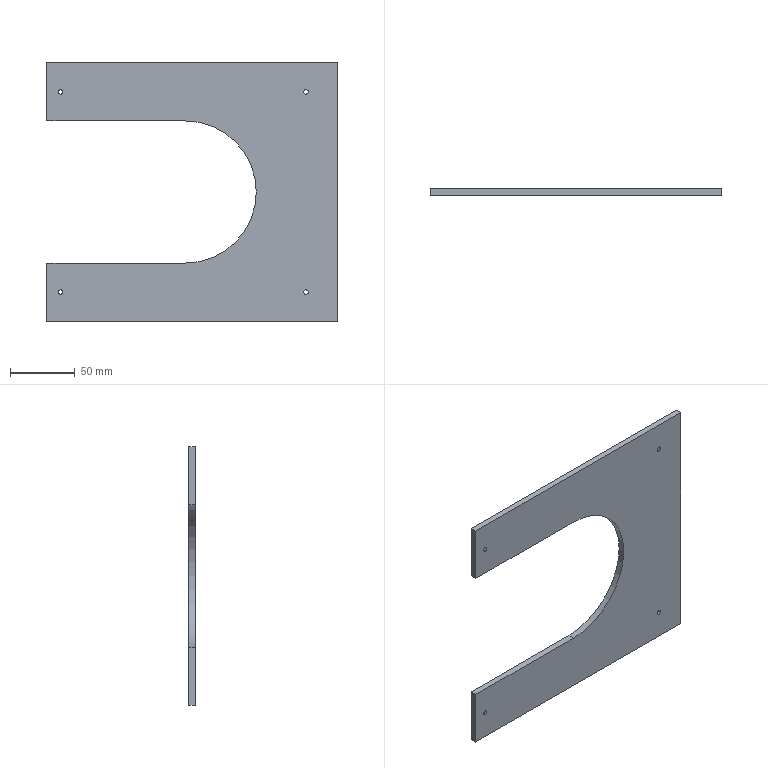CAM job | Mastercam | mm | 4 operations | part box 224.5 x 5 x 200
1. Contour (Ramp) | 3 - 3 平铣刀
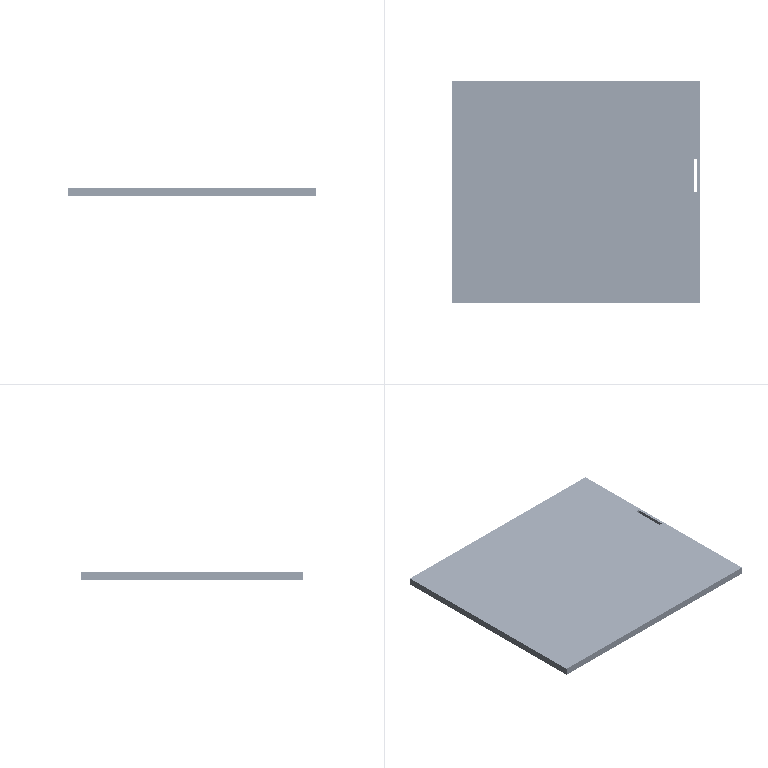2. Drill/Counterbore | 7 - 4 倒角刀
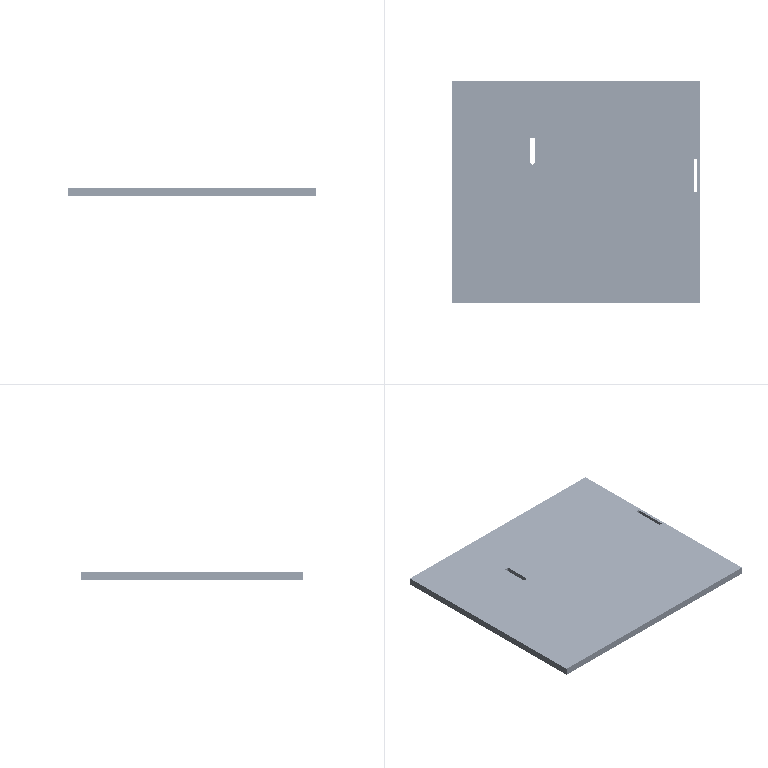3. Contour (2D chamfer) | 7 - 4 倒角刀
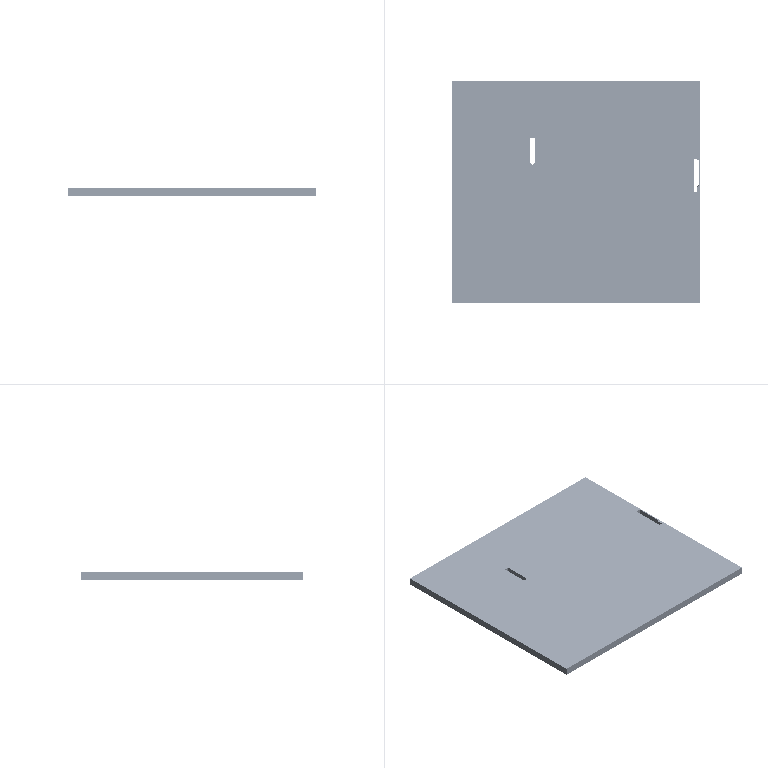4. Contour (Ramp) | 2 - 2 平铣刀